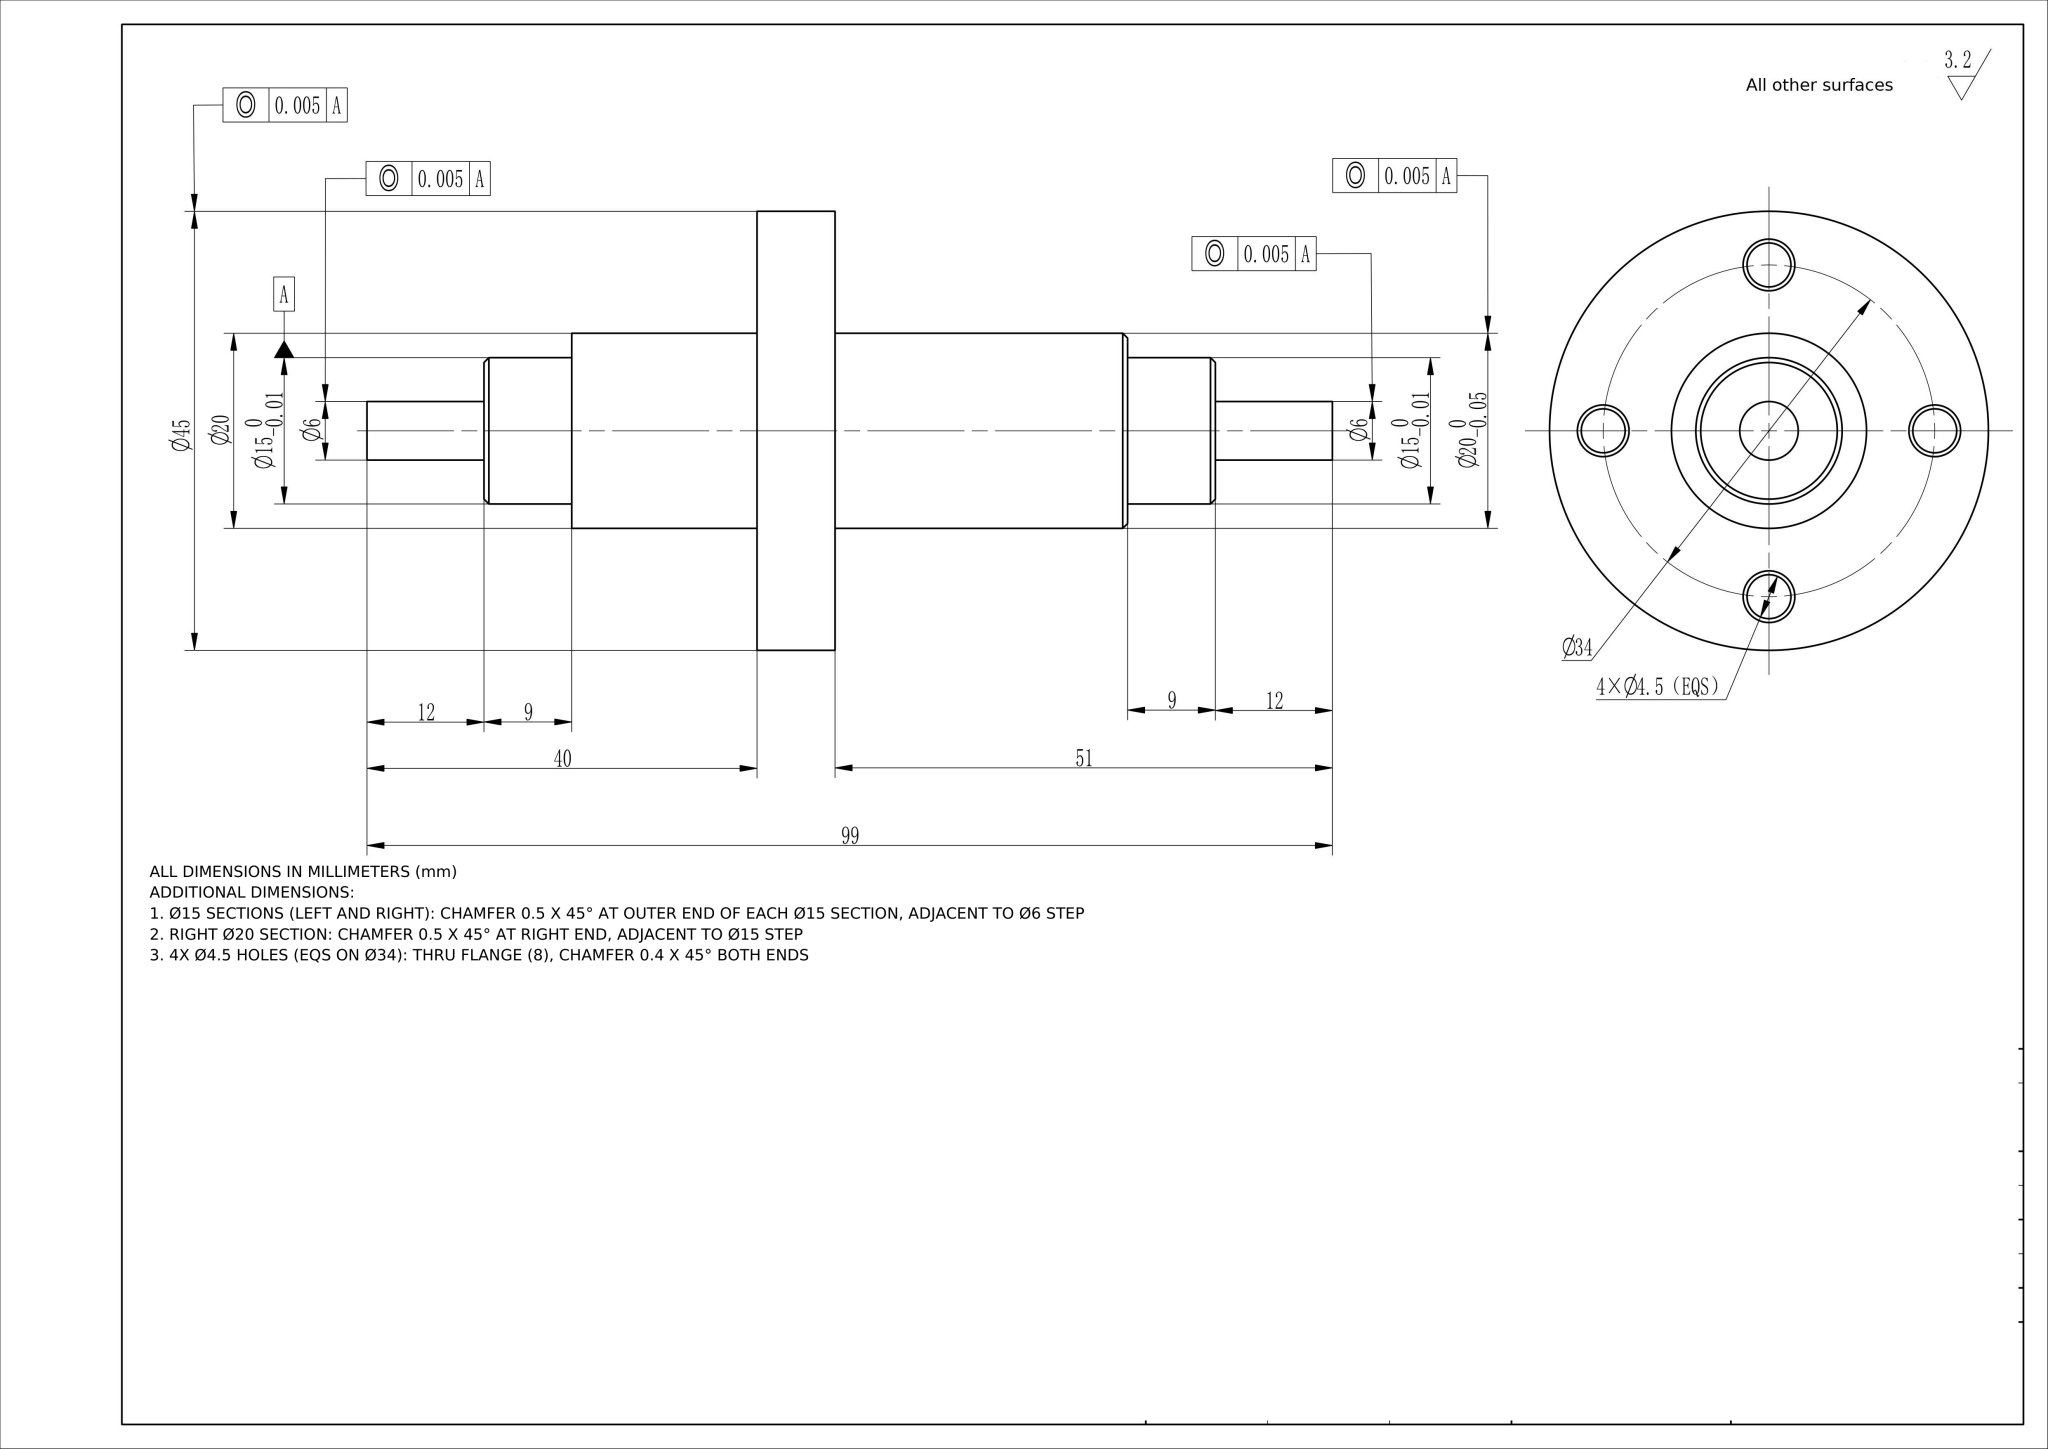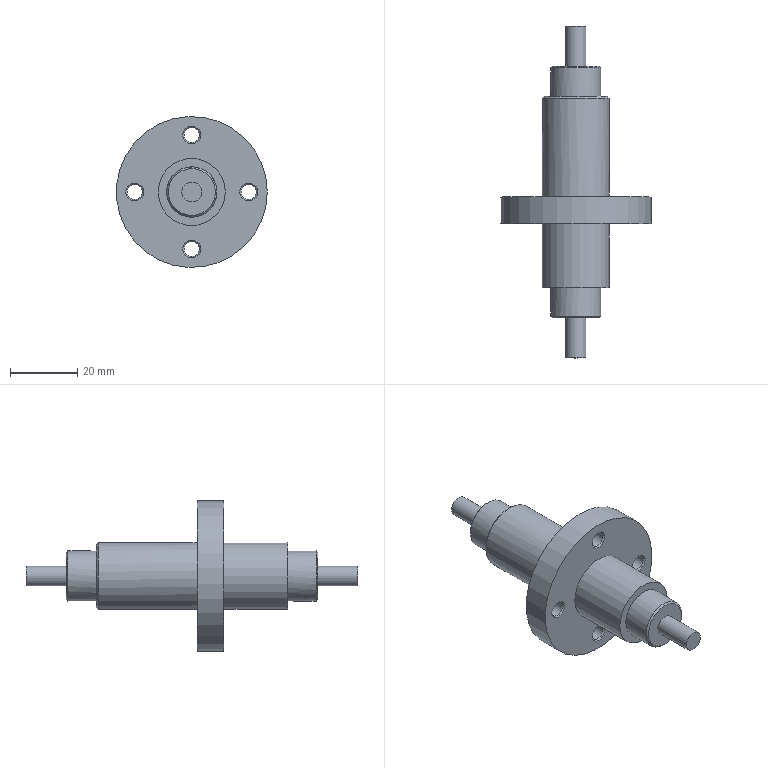Part | NX | mm | 1 solid | 30 faces | box 45 x 99 x 45 mm | volume 31439 mm3 | cylinder 11 | cone 11 | plane 8 | commonest cylinder face diameters 4.5 x4 20 x2 15 x2 6 x2 45 x1
STEP:
#1=CARTESIAN_POINT('',(0.,0.,0.));
#2=DIRECTION('',(0.,0.,1.));
#3=DIRECTION('',(1.,0.,0.));
#4=AXIS2_PLACEMENT_3D('',#1,#2,#3);
#5=(LENGTH_UNIT()NAMED_UNIT(*)SI_UNIT(.MILLI.,.METRE.));
#6=UNCERTAINTY_MEASURE_WITH_UNIT(LENGTH_MEASURE(0.00002),#5,'','');
#7=(NAMED_UNIT(*)PLANE_ANGLE_UNIT()SI_UNIT($,.RADIAN.));
#8=PLANE_ANGLE_MEASURE_WITH_UNIT(PLANE_ANGLE_MEASURE(0.01745),#7);
#9=DIMENSIONAL_EXPONENTS(0.,0.,0.,0.,0.,0.,0.);
#10=(CONVERSION_BASED_UNIT('',#8)NAMED_UNIT(#9)PLANE_ANGLE_UNIT());
#11=(NAMED_UNIT(*)SI_UNIT($,.STERADIAN.)SOLID_ANGLE_UNIT());
#12=(GEOMETRIC_REPRESENTATION_CONTEXT(3)GLOBAL_UNCERTAINTY_ASSIGNED_CONTEXT((#6))GLOBAL_UNIT_ASSIGNED_CONTEXT((#5,#10,#11))REPRESENTATION_CONTEXT('',''));
#13=SHAPE_REPRESENTATION('',(#4),#12);
#14=CARTESIAN_POINT('',(0.,29.5,-10.));
#15=VERTEX_POINT('',#14);
#16=CARTESIAN_POINT('',(0.,29.5,0.));
#17=DIRECTION('',(0.,-1.,0.));
#18=DIRECTION('',(0.,0.,-1.));
#19=AXIS2_PLACEMENT_3D('',#16,#17,#18);
#20=CIRCLE('',#19,10.);
#21=EDGE_CURVE('',#15,#15,#20,.T.);
#22=ORIENTED_EDGE('',*,*,#21,.T.);
#23=EDGE_LOOP('',(#22));
#24=FACE_BOUND('',#23,.T.);
#25=CARTESIAN_POINT('',(10.,0.,-0.));
#26=VERTEX_POINT('',#25);
#27=CARTESIAN_POINT('',(0.,0.,0.));
#28=DIRECTION('',(0.,-1.,0.));
#29=DIRECTION('',(1.,0.,-0.));
#30=AXIS2_PLACEMENT_3D('',#27,#28,#29);
#31=CIRCLE('',#30,10.);
#32=EDGE_CURVE('',#26,#26,#31,.T.);
#33=ORIENTED_EDGE('',*,*,#32,.F.);
#34=EDGE_LOOP('',(#33));
#35=FACE_BOUND('',#34,.T.);
#36=CARTESIAN_POINT('',(0.,30.,0.));
#37=DIRECTION('',(0.,-1.,0.));
#38=DIRECTION('',(0.,0.,-1.));
#39=AXIS2_PLACEMENT_3D('',#36,#37,#38);
#40=CYLINDRICAL_SURFACE('',#39,10.);
#41=ADVANCED_FACE('',(#24,#35),#40,.T.);
#42=CARTESIAN_POINT('',(0.,30.,-9.5));
#43=VERTEX_POINT('',#42);
#44=CARTESIAN_POINT('',(0.,30.,0.));
#45=DIRECTION('',(0.,1.,0.));
#46=DIRECTION('',(0.,0.,-1.));
#47=AXIS2_PLACEMENT_3D('',#44,#45,#46);
#48=CIRCLE('',#47,9.5);
#49=EDGE_CURVE('',#43,#43,#48,.T.);
#50=ORIENTED_EDGE('',*,*,#49,.T.);
#51=EDGE_LOOP('',(#50));
#52=FACE_BOUND('',#51,.T.);
#53=CARTESIAN_POINT('',(7.5,30.,0.));
#54=VERTEX_POINT('',#53);
#55=CARTESIAN_POINT('',(0.,30.,0.));
#56=DIRECTION('',(0.,1.,0.));
#57=DIRECTION('',(1.,0.,0.));
#58=AXIS2_PLACEMENT_3D('',#55,#56,#57);
#59=CIRCLE('',#58,7.5);
#60=EDGE_CURVE('',#54,#54,#59,.T.);
#61=ORIENTED_EDGE('',*,*,#60,.F.);
#62=EDGE_LOOP('',(#61));
#63=FACE_BOUND('',#62,.T.);
#64=CARTESIAN_POINT('',(0.,30.,0.));
#65=DIRECTION('',(0.,-1.,0.));
#66=DIRECTION('',(0.,0.,-1.));
#67=AXIS2_PLACEMENT_3D('',#64,#65,#66);
#68=PLANE('',#67);
#69=ADVANCED_FACE('',(#52,#63),#68,.F.);
#70=CARTESIAN_POINT('',(22.5,-8.,-0.));
#71=VERTEX_POINT('',#70);
#72=CARTESIAN_POINT('',(0.,-8.,0.));
#73=DIRECTION('',(0.,-1.,0.));
#74=DIRECTION('',(1.,0.,-0.));
#75=AXIS2_PLACEMENT_3D('',#72,#73,#74);
#76=CIRCLE('',#75,22.5);
#77=EDGE_CURVE('',#71,#71,#76,.T.);
#78=ORIENTED_EDGE('',*,*,#77,.F.);
#79=EDGE_LOOP('',(#78));
#80=FACE_BOUND('',#79,.T.);
#81=CARTESIAN_POINT('',(22.5,0.,-0.));
#82=VERTEX_POINT('',#81);
#83=CARTESIAN_POINT('',(0.,0.,0.));
#84=DIRECTION('',(0.,-1.,0.));
#85=DIRECTION('',(1.,0.,-0.));
#86=AXIS2_PLACEMENT_3D('',#83,#84,#85);
#87=CIRCLE('',#86,22.5);
#88=EDGE_CURVE('',#82,#82,#87,.T.);
#89=ORIENTED_EDGE('',*,*,#88,.T.);
#90=EDGE_LOOP('',(#89));
#91=FACE_BOUND('',#90,.T.);
#92=CARTESIAN_POINT('',(0.,-8.,0.));
#93=DIRECTION('',(0.,1.,0.));
#94=DIRECTION('',(0.,0.,1.));
#95=AXIS2_PLACEMENT_3D('',#92,#93,#94);
#96=CYLINDRICAL_SURFACE('',#95,22.5);
#97=ADVANCED_FACE('',(#80,#91),#96,.T.);
#98=CARTESIAN_POINT('',(17.,-8.,-2.65));
#99=VERTEX_POINT('',#98);
#100=CARTESIAN_POINT('',(17.,-8.,0.));
#101=DIRECTION('',(0.,1.,0.));
#102=DIRECTION('',(0.,0.,-1.));
#103=AXIS2_PLACEMENT_3D('',#100,#101,#102);
#104=CIRCLE('',#103,2.65);
#105=EDGE_CURVE('',#99,#99,#104,.T.);
#106=ORIENTED_EDGE('',*,*,#105,.T.);
#107=EDGE_LOOP('',(#106));
#108=FACE_BOUND('',#107,.T.);
#109=CARTESIAN_POINT('',(0.,-8.,14.35));
#110=VERTEX_POINT('',#109);
#111=CARTESIAN_POINT('',(0.,-8.,17.));
#112=DIRECTION('',(0.,1.,0.));
#113=DIRECTION('',(0.,0.,-1.));
#114=AXIS2_PLACEMENT_3D('',#111,#112,#113);
#115=CIRCLE('',#114,2.65);
#116=EDGE_CURVE('',#110,#110,#115,.T.);
#117=ORIENTED_EDGE('',*,*,#116,.T.);
#118=EDGE_LOOP('',(#117));
#119=FACE_BOUND('',#118,.T.);
#120=CARTESIAN_POINT('',(0.,-8.,-19.65));
#121=VERTEX_POINT('',#120);
#122=CARTESIAN_POINT('',(0.,-8.,-17.));
#123=DIRECTION('',(0.,1.,0.));
#124=DIRECTION('',(0.,0.,-1.));
#125=AXIS2_PLACEMENT_3D('',#122,#123,#124);
#126=CIRCLE('',#125,2.65);
#127=EDGE_CURVE('',#121,#121,#126,.T.);
#128=ORIENTED_EDGE('',*,*,#127,.T.);
#129=EDGE_LOOP('',(#128));
#130=FACE_BOUND('',#129,.T.);
#131=CARTESIAN_POINT('',(-17.,-8.,-2.65));
#132=VERTEX_POINT('',#131);
#133=CARTESIAN_POINT('',(-17.,-8.,0.));
#134=DIRECTION('',(0.,1.,0.));
#135=DIRECTION('',(0.,0.,-1.));
#136=AXIS2_PLACEMENT_3D('',#133,#134,#135);
#137=CIRCLE('',#136,2.65);
#138=EDGE_CURVE('',#132,#132,#137,.T.);
#139=ORIENTED_EDGE('',*,*,#138,.T.);
#140=EDGE_LOOP('',(#139));
#141=FACE_BOUND('',#140,.T.);
#142=CARTESIAN_POINT('',(10.,-8.,-0.));
#143=VERTEX_POINT('',#142);
#144=CARTESIAN_POINT('',(0.,-8.,0.));
#145=DIRECTION('',(0.,-1.,0.));
#146=DIRECTION('',(1.,0.,-0.));
#147=AXIS2_PLACEMENT_3D('',#144,#145,#146);
#148=CIRCLE('',#147,10.);
#149=EDGE_CURVE('',#143,#143,#148,.T.);
#150=ORIENTED_EDGE('',*,*,#149,.F.);
#151=EDGE_LOOP('',(#150));
#152=FACE_BOUND('',#151,.T.);
#153=ORIENTED_EDGE('',*,*,#77,.T.);
#154=EDGE_LOOP('',(#153));
#155=FACE_BOUND('',#154,.T.);
#156=CARTESIAN_POINT('',(0.,-8.,0.));
#157=DIRECTION('',(0.,-1.,0.));
#158=DIRECTION('',(0.,0.,-1.));
#159=AXIS2_PLACEMENT_3D('',#156,#157,#158);
#160=PLANE('',#159);
#161=ADVANCED_FACE('',(#108,#119,#130,#141,#152,#155),#160,.T.);
#162=CARTESIAN_POINT('',(17.,0.,-2.65));
#163=VERTEX_POINT('',#162);
#164=CARTESIAN_POINT('',(17.,0.,0.));
#165=DIRECTION('',(0.,-1.,0.));
#166=DIRECTION('',(0.,0.,-1.));
#167=AXIS2_PLACEMENT_3D('',#164,#165,#166);
#168=CIRCLE('',#167,2.65);
#169=EDGE_CURVE('',#163,#163,#168,.T.);
#170=ORIENTED_EDGE('',*,*,#169,.T.);
#171=EDGE_LOOP('',(#170));
#172=FACE_BOUND('',#171,.T.);
#173=CARTESIAN_POINT('',(0.,0.,14.35));
#174=VERTEX_POINT('',#173);
#175=CARTESIAN_POINT('',(0.,0.,17.));
#176=DIRECTION('',(0.,-1.,0.));
#177=DIRECTION('',(0.,0.,-1.));
#178=AXIS2_PLACEMENT_3D('',#175,#176,#177);
#179=CIRCLE('',#178,2.65);
#180=EDGE_CURVE('',#174,#174,#179,.T.);
#181=ORIENTED_EDGE('',*,*,#180,.T.);
#182=EDGE_LOOP('',(#181));
#183=FACE_BOUND('',#182,.T.);
#184=CARTESIAN_POINT('',(0.,0.,-19.65));
#185=VERTEX_POINT('',#184);
#186=CARTESIAN_POINT('',(0.,0.,-17.));
#187=DIRECTION('',(0.,-1.,0.));
#188=DIRECTION('',(0.,0.,-1.));
#189=AXIS2_PLACEMENT_3D('',#186,#187,#188);
#190=CIRCLE('',#189,2.65);
#191=EDGE_CURVE('',#185,#185,#190,.T.);
#192=ORIENTED_EDGE('',*,*,#191,.T.);
#193=EDGE_LOOP('',(#192));
#194=FACE_BOUND('',#193,.T.);
#195=CARTESIAN_POINT('',(-17.,0.,-2.65));
#196=VERTEX_POINT('',#195);
#197=CARTESIAN_POINT('',(-17.,0.,0.));
#198=DIRECTION('',(0.,-1.,0.));
#199=DIRECTION('',(0.,0.,-1.));
#200=AXIS2_PLACEMENT_3D('',#197,#198,#199);
#201=CIRCLE('',#200,2.65);
#202=EDGE_CURVE('',#196,#196,#201,.T.);
#203=ORIENTED_EDGE('',*,*,#202,.T.);
#204=EDGE_LOOP('',(#203));
#205=FACE_BOUND('',#204,.T.);
#206=ORIENTED_EDGE('',*,*,#32,.T.);
#207=EDGE_LOOP('',(#206));
#208=FACE_BOUND('',#207,.T.);
#209=ORIENTED_EDGE('',*,*,#88,.F.);
#210=EDGE_LOOP('',(#209));
#211=FACE_BOUND('',#210,.T.);
#212=CARTESIAN_POINT('',(0.,0.,0.));
#213=DIRECTION('',(0.,-1.,0.));
#214=DIRECTION('',(0.,0.,-1.));
#215=AXIS2_PLACEMENT_3D('',#212,#213,#214);
#216=PLANE('',#215);
#217=ADVANCED_FACE('',(#172,#183,#194,#205,#208,#211),#216,.F.);
#218=CARTESIAN_POINT('',(0.,38.5,7.5));
#219=VERTEX_POINT('',#218);
#220=CARTESIAN_POINT('',(0.,38.5,0.));
#221=DIRECTION('',(0.,-1.,0.));
#222=DIRECTION('',(0.,0.,1.));
#223=AXIS2_PLACEMENT_3D('',#220,#221,#222);
#224=CIRCLE('',#223,7.5);
#225=EDGE_CURVE('',#219,#219,#224,.T.);
#226=ORIENTED_EDGE('',*,*,#225,.T.);
#227=EDGE_LOOP('',(#226));
#228=FACE_BOUND('',#227,.T.);
#229=ORIENTED_EDGE('',*,*,#60,.T.);
#230=EDGE_LOOP('',(#229));
#231=FACE_BOUND('',#230,.T.);
#232=CARTESIAN_POINT('',(0.,39.,0.));
#233=DIRECTION('',(0.,-1.,0.));
#234=DIRECTION('',(0.,0.,-1.));
#235=AXIS2_PLACEMENT_3D('',#232,#233,#234);
#236=CYLINDRICAL_SURFACE('',#235,7.5);
#237=ADVANCED_FACE('',(#228,#231),#236,.T.);
#238=CARTESIAN_POINT('',(0.,39.,7.));
#239=VERTEX_POINT('',#238);
#240=CARTESIAN_POINT('',(0.,39.,0.));
#241=DIRECTION('',(0.,1.,0.));
#242=DIRECTION('',(0.,0.,1.));
#243=AXIS2_PLACEMENT_3D('',#240,#241,#242);
#244=CIRCLE('',#243,7.);
#245=EDGE_CURVE('',#239,#239,#244,.T.);
#246=ORIENTED_EDGE('',*,*,#245,.T.);
#247=EDGE_LOOP('',(#246));
#248=FACE_BOUND('',#247,.T.);
#249=CARTESIAN_POINT('',(3.,39.,0.));
#250=VERTEX_POINT('',#249);
#251=CARTESIAN_POINT('',(0.,39.,0.));
#252=DIRECTION('',(0.,1.,0.));
#253=DIRECTION('',(1.,0.,0.));
#254=AXIS2_PLACEMENT_3D('',#251,#252,#253);
#255=CIRCLE('',#254,3.);
#256=EDGE_CURVE('',#250,#250,#255,.T.);
#257=ORIENTED_EDGE('',*,*,#256,.F.);
#258=EDGE_LOOP('',(#257));
#259=FACE_BOUND('',#258,.T.);
#260=CARTESIAN_POINT('',(0.,39.,0.));
#261=DIRECTION('',(0.,1.,0.));
#262=DIRECTION('',(0.,0.,1.));
#263=AXIS2_PLACEMENT_3D('',#260,#261,#262);
#264=PLANE('',#263);
#265=ADVANCED_FACE('',(#248,#259),#264,.T.);
#266=CARTESIAN_POINT('',(10.,-27.,-0.));
#267=VERTEX_POINT('',#266);
#268=CARTESIAN_POINT('',(0.,-27.,0.));
#269=DIRECTION('',(0.,-1.,0.));
#270=DIRECTION('',(1.,0.,-0.));
#271=AXIS2_PLACEMENT_3D('',#268,#269,#270);
#272=CIRCLE('',#271,10.);
#273=EDGE_CURVE('',#267,#267,#272,.T.);
#274=ORIENTED_EDGE('',*,*,#273,.F.);
#275=EDGE_LOOP('',(#274));
#276=FACE_BOUND('',#275,.T.);
#277=ORIENTED_EDGE('',*,*,#149,.T.);
#278=EDGE_LOOP('',(#277));
#279=FACE_BOUND('',#278,.T.);
#280=CARTESIAN_POINT('',(0.,-27.,0.));
#281=DIRECTION('',(0.,1.,0.));
#282=DIRECTION('',(0.,0.,1.));
#283=AXIS2_PLACEMENT_3D('',#280,#281,#282);
#284=CYLINDRICAL_SURFACE('',#283,10.);
#285=ADVANCED_FACE('',(#276,#279),#284,.T.);
#286=CARTESIAN_POINT('',(7.5,-27.,-0.));
#287=VERTEX_POINT('',#286);
#288=CARTESIAN_POINT('',(0.,-27.,0.));
#289=DIRECTION('',(0.,-1.,0.));
#290=DIRECTION('',(1.,0.,-0.));
#291=AXIS2_PLACEMENT_3D('',#288,#289,#290);
#292=CIRCLE('',#291,7.5);
#293=EDGE_CURVE('',#287,#287,#292,.T.);
#294=ORIENTED_EDGE('',*,*,#293,.F.);
#295=EDGE_LOOP('',(#294));
#296=FACE_BOUND('',#295,.T.);
#297=ORIENTED_EDGE('',*,*,#273,.T.);
#298=EDGE_LOOP('',(#297));
#299=FACE_BOUND('',#298,.T.);
#300=CARTESIAN_POINT('',(0.,-27.,0.));
#301=DIRECTION('',(0.,-1.,0.));
#302=DIRECTION('',(0.,0.,-1.));
#303=AXIS2_PLACEMENT_3D('',#300,#301,#302);
#304=PLANE('',#303);
#305=ADVANCED_FACE('',(#296,#299),#304,.T.);
#306=CARTESIAN_POINT('',(0.,-35.5,-7.5));
#307=VERTEX_POINT('',#306);
#308=CARTESIAN_POINT('',(0.,-35.5,0.));
#309=DIRECTION('',(0.,1.,0.));
#310=DIRECTION('',(0.,0.,-1.));
#311=AXIS2_PLACEMENT_3D('',#308,#309,#310);
#312=CIRCLE('',#311,7.5);
#313=EDGE_CURVE('',#307,#307,#312,.T.);
#314=ORIENTED_EDGE('',*,*,#313,.T.);
#315=EDGE_LOOP('',(#314));
#316=FACE_BOUND('',#315,.T.);
#317=ORIENTED_EDGE('',*,*,#293,.T.);
#318=EDGE_LOOP('',(#317));
#319=FACE_BOUND('',#318,.T.);
#320=CARTESIAN_POINT('',(0.,-36.,0.));
#321=DIRECTION('',(0.,1.,0.));
#322=DIRECTION('',(0.,0.,1.));
#323=AXIS2_PLACEMENT_3D('',#320,#321,#322);
#324=CYLINDRICAL_SURFACE('',#323,7.5);
#325=ADVANCED_FACE('',(#316,#319),#324,.T.);
#326=CARTESIAN_POINT('',(0.,-36.,-7.));
#327=VERTEX_POINT('',#326);
#328=CARTESIAN_POINT('',(0.,-36.,0.));
#329=DIRECTION('',(0.,-1.,0.));
#330=DIRECTION('',(0.,0.,-1.));
#331=AXIS2_PLACEMENT_3D('',#328,#329,#330);
#332=CIRCLE('',#331,7.);
#333=EDGE_CURVE('',#327,#327,#332,.T.);
#334=ORIENTED_EDGE('',*,*,#333,.T.);
#335=EDGE_LOOP('',(#334));
#336=FACE_BOUND('',#335,.T.);
#337=CARTESIAN_POINT('',(3.,-36.,-0.));
#338=VERTEX_POINT('',#337);
#339=CARTESIAN_POINT('',(0.,-36.,0.));
#340=DIRECTION('',(0.,-1.,0.));
#341=DIRECTION('',(1.,0.,-0.));
#342=AXIS2_PLACEMENT_3D('',#339,#340,#341);
#343=CIRCLE('',#342,3.);
#344=EDGE_CURVE('',#338,#338,#343,.T.);
#345=ORIENTED_EDGE('',*,*,#344,.F.);
#346=EDGE_LOOP('',(#345));
#347=FACE_BOUND('',#346,.T.);
#348=CARTESIAN_POINT('',(0.,-36.,0.));
#349=DIRECTION('',(0.,-1.,0.));
#350=DIRECTION('',(0.,0.,-1.));
#351=AXIS2_PLACEMENT_3D('',#348,#349,#350);
#352=PLANE('',#351);
#353=ADVANCED_FACE('',(#336,#347),#352,.T.);
#354=CARTESIAN_POINT('',(-17.,-0.4,-2.25));
#355=VERTEX_POINT('',#354);
#356=CARTESIAN_POINT('',(-17.,-0.4,0.));
#357=DIRECTION('',(0.,1.,0.));
#358=DIRECTION('',(0.,0.,-1.));
#359=AXIS2_PLACEMENT_3D('',#356,#357,#358);
#360=CIRCLE('',#359,2.25);
#361=EDGE_CURVE('',#355,#355,#360,.T.);
#362=ORIENTED_EDGE('',*,*,#361,.T.);
#363=EDGE_LOOP('',(#362));
#364=FACE_BOUND('',#363,.T.);
#365=CARTESIAN_POINT('',(-17.,-7.6,-2.25));
#366=VERTEX_POINT('',#365);
#367=CARTESIAN_POINT('',(-17.,-7.6,0.));
#368=DIRECTION('',(0.,-1.,0.));
#369=DIRECTION('',(0.,0.,-1.));
#370=AXIS2_PLACEMENT_3D('',#367,#368,#369);
#371=CIRCLE('',#370,2.25);
#372=EDGE_CURVE('',#366,#366,#371,.T.);
#373=ORIENTED_EDGE('',*,*,#372,.T.);
#374=EDGE_LOOP('',(#373));
#375=FACE_BOUND('',#374,.T.);
#376=CARTESIAN_POINT('',(-17.,-8.,0.));
#377=DIRECTION('',(0.,1.,0.));
#378=DIRECTION('',(0.,0.,1.));
#379=AXIS2_PLACEMENT_3D('',#376,#377,#378);
#380=CYLINDRICAL_SURFACE('',#379,2.25);
#381=ADVANCED_FACE('',(#364,#375),#380,.F.);
#382=ORIENTED_EDGE('',*,*,#372,.F.);
#383=EDGE_LOOP('',(#382));
#384=FACE_BOUND('',#383,.T.);
#385=ORIENTED_EDGE('',*,*,#138,.F.);
#386=EDGE_LOOP('',(#385));
#387=FACE_BOUND('',#386,.T.);
#388=CARTESIAN_POINT('',(-17.,-8.,0.));
#389=DIRECTION('',(0.,-1.,0.));
#390=DIRECTION('',(0.,0.,-1.));
#391=AXIS2_PLACEMENT_3D('',#388,#389,#390);
#392=CONICAL_SURFACE('',#391,2.65,45.);
#393=ADVANCED_FACE('',(#384,#387),#392,.F.);
#394=ORIENTED_EDGE('',*,*,#202,.F.);
#395=EDGE_LOOP('',(#394));
#396=FACE_BOUND('',#395,.T.);
#397=ORIENTED_EDGE('',*,*,#361,.F.);
#398=EDGE_LOOP('',(#397));
#399=FACE_BOUND('',#398,.T.);
#400=CARTESIAN_POINT('',(-17.,-0.4,0.));
#401=DIRECTION('',(0.,1.,0.));
#402=DIRECTION('',(0.,0.,1.));
#403=AXIS2_PLACEMENT_3D('',#400,#401,#402);
#404=CONICAL_SURFACE('',#403,2.25,45.);
#405=ADVANCED_FACE('',(#396,#399),#404,.F.);
#406=CARTESIAN_POINT('',(0.,-0.4,-19.25));
#407=VERTEX_POINT('',#406);
#408=CARTESIAN_POINT('',(0.,-0.4,-17.));
#409=DIRECTION('',(0.,1.,0.));
#410=DIRECTION('',(0.,0.,-1.));
#411=AXIS2_PLACEMENT_3D('',#408,#409,#410);
#412=CIRCLE('',#411,2.25);
#413=EDGE_CURVE('',#407,#407,#412,.T.);
#414=ORIENTED_EDGE('',*,*,#413,.T.);
#415=EDGE_LOOP('',(#414));
#416=FACE_BOUND('',#415,.T.);
#417=CARTESIAN_POINT('',(0.,-7.6,-19.25));
#418=VERTEX_POINT('',#417);
#419=CARTESIAN_POINT('',(0.,-7.6,-17.));
#420=DIRECTION('',(0.,-1.,0.));
#421=DIRECTION('',(0.,0.,-1.));
#422=AXIS2_PLACEMENT_3D('',#419,#420,#421);
#423=CIRCLE('',#422,2.25);
#424=EDGE_CURVE('',#418,#418,#423,.T.);
#425=ORIENTED_EDGE('',*,*,#424,.T.);
#426=EDGE_LOOP('',(#425));
#427=FACE_BOUND('',#426,.T.);
#428=CARTESIAN_POINT('',(0.,-8.,-17.));
#429=DIRECTION('',(0.,1.,0.));
#430=DIRECTION('',(0.,0.,1.));
#431=AXIS2_PLACEMENT_3D('',#428,#429,#430);
#432=CYLINDRICAL_SURFACE('',#431,2.25);
#433=ADVANCED_FACE('',(#416,#427),#432,.F.);
#434=ORIENTED_EDGE('',*,*,#424,.F.);
#435=EDGE_LOOP('',(#434));
#436=FACE_BOUND('',#435,.T.);
#437=ORIENTED_EDGE('',*,*,#127,.F.);
#438=EDGE_LOOP('',(#437));
#439=FACE_BOUND('',#438,.T.);
#440=CARTESIAN_POINT('',(0.,-8.,-17.));
#441=DIRECTION('',(0.,-1.,0.));
#442=DIRECTION('',(0.,0.,-1.));
#443=AXIS2_PLACEMENT_3D('',#440,#441,#442);
#444=CONICAL_SURFACE('',#443,2.65,45.);
#445=ADVANCED_FACE('',(#436,#439),#444,.F.);
#446=ORIENTED_EDGE('',*,*,#191,.F.);
#447=EDGE_LOOP('',(#446));
#448=FACE_BOUND('',#447,.T.);
#449=ORIENTED_EDGE('',*,*,#413,.F.);
#450=EDGE_LOOP('',(#449));
#451=FACE_BOUND('',#450,.T.);
#452=CARTESIAN_POINT('',(0.,-0.4,-17.));
#453=DIRECTION('',(0.,1.,0.));
#454=DIRECTION('',(0.,0.,1.));
#455=AXIS2_PLACEMENT_3D('',#452,#453,#454);
#456=CONICAL_SURFACE('',#455,2.25,45.);
#457=ADVANCED_FACE('',(#448,#451),#456,.F.);
#458=CARTESIAN_POINT('',(0.,-0.4,14.75));
#459=VERTEX_POINT('',#458);
#460=CARTESIAN_POINT('',(0.,-0.4,17.));
#461=DIRECTION('',(0.,1.,0.));
#462=DIRECTION('',(0.,0.,-1.));
#463=AXIS2_PLACEMENT_3D('',#460,#461,#462);
#464=CIRCLE('',#463,2.25);
#465=EDGE_CURVE('',#459,#459,#464,.T.);
#466=ORIENTED_EDGE('',*,*,#465,.T.);
#467=EDGE_LOOP('',(#466));
#468=FACE_BOUND('',#467,.T.);
#469=CARTESIAN_POINT('',(0.,-7.6,14.75));
#470=VERTEX_POINT('',#469);
#471=CARTESIAN_POINT('',(0.,-7.6,17.));
#472=DIRECTION('',(0.,-1.,0.));
#473=DIRECTION('',(0.,0.,-1.));
#474=AXIS2_PLACEMENT_3D('',#471,#472,#473);
#475=CIRCLE('',#474,2.25);
#476=EDGE_CURVE('',#470,#470,#475,.T.);
#477=ORIENTED_EDGE('',*,*,#476,.T.);
#478=EDGE_LOOP('',(#477));
#479=FACE_BOUND('',#478,.T.);
#480=CARTESIAN_POINT('',(0.,-8.,17.));
#481=DIRECTION('',(0.,1.,0.));
#482=DIRECTION('',(0.,0.,1.));
#483=AXIS2_PLACEMENT_3D('',#480,#481,#482);
#484=CYLINDRICAL_SURFACE('',#483,2.25);
#485=ADVANCED_FACE('',(#468,#479),#484,.F.);
#486=ORIENTED_EDGE('',*,*,#476,.F.);
#487=EDGE_LOOP('',(#486));
#488=FACE_BOUND('',#487,.T.);
#489=ORIENTED_EDGE('',*,*,#116,.F.);
#490=EDGE_LOOP('',(#489));
#491=FACE_BOUND('',#490,.T.);
#492=CARTESIAN_POINT('',(0.,-8.,17.));
#493=DIRECTION('',(0.,-1.,0.));
#494=DIRECTION('',(0.,0.,-1.));
#495=AXIS2_PLACEMENT_3D('',#492,#493,#494);
#496=CONICAL_SURFACE('',#495,2.65,45.);
#497=ADVANCED_FACE('',(#488,#491),#496,.F.);
#498=ORIENTED_EDGE('',*,*,#180,.F.);
#499=EDGE_LOOP('',(#498));
#500=FACE_BOUND('',#499,.T.);
#501=ORIENTED_EDGE('',*,*,#465,.F.);
#502=EDGE_LOOP('',(#501));
#503=FACE_BOUND('',#502,.T.);
#504=CARTESIAN_POINT('',(0.,-0.4,17.));
#505=DIRECTION('',(0.,1.,0.));
#506=DIRECTION('',(0.,0.,1.));
#507=AXIS2_PLACEMENT_3D('',#504,#505,#506);
#508=CONICAL_SURFACE('',#507,2.25,45.);
#509=ADVANCED_FACE('',(#500,#503),#508,.F.);
#510=CARTESIAN_POINT('',(17.,-0.4,-2.25));
#511=VERTEX_POINT('',#510);
#512=CARTESIAN_POINT('',(17.,-0.4,0.));
#513=DIRECTION('',(0.,1.,0.));
#514=DIRECTION('',(0.,0.,-1.));
#515=AXIS2_PLACEMENT_3D('',#512,#513,#514);
#516=CIRCLE('',#515,2.25);
#517=EDGE_CURVE('',#511,#511,#516,.T.);
#518=ORIENTED_EDGE('',*,*,#517,.T.);
#519=EDGE_LOOP('',(#518));
#520=FACE_BOUND('',#519,.T.);
#521=CARTESIAN_POINT('',(17.,-7.6,-2.25));
#522=VERTEX_POINT('',#521);
#523=CARTESIAN_POINT('',(17.,-7.6,0.));
#524=DIRECTION('',(0.,-1.,0.));
#525=DIRECTION('',(0.,0.,-1.));
#526=AXIS2_PLACEMENT_3D('',#523,#524,#525);
#527=CIRCLE('',#526,2.25);
#528=EDGE_CURVE('',#522,#522,#527,.T.);
#529=ORIENTED_EDGE('',*,*,#528,.T.);
#530=EDGE_LOOP('',(#529));
#531=FACE_BOUND('',#530,.T.);
#532=CARTESIAN_POINT('',(17.,-8.,0.));
#533=DIRECTION('',(0.,1.,0.));
#534=DIRECTION('',(0.,0.,1.));
#535=AXIS2_PLACEMENT_3D('',#532,#533,#534);
#536=CYLINDRICAL_SURFACE('',#535,2.25);
#537=ADVANCED_FACE('',(#520,#531),#536,.F.);
#538=ORIENTED_EDGE('',*,*,#528,.F.);
#539=EDGE_LOOP('',(#538));
#540=FACE_BOUND('',#539,.T.);
#541=ORIENTED_EDGE('',*,*,#105,.F.);
#542=EDGE_LOOP('',(#541));
#543=FACE_BOUND('',#542,.T.);
#544=CARTESIAN_POINT('',(17.,-8.,0.));
#545=DIRECTION('',(0.,-1.,0.));
#546=DIRECTION('',(0.,0.,-1.));
#547=AXIS2_PLACEMENT_3D('',#544,#545,#546);
#548=CONICAL_SURFACE('',#547,2.65,45.);
#549=ADVANCED_FACE('',(#540,#543),#548,.F.);
#550=ORIENTED_EDGE('',*,*,#169,.F.);
#551=EDGE_LOOP('',(#550));
#552=FACE_BOUND('',#551,.T.);
#553=ORIENTED_EDGE('',*,*,#517,.F.);
#554=EDGE_LOOP('',(#553));
#555=FACE_BOUND('',#554,.T.);
#556=CARTESIAN_POINT('',(17.,-0.4,0.));
#557=DIRECTION('',(0.,1.,0.));
#558=DIRECTION('',(0.,0.,1.));
#559=AXIS2_PLACEMENT_3D('',#556,#557,#558);
#560=CONICAL_SURFACE('',#559,2.25,45.);
#561=ADVANCED_FACE('',(#552,#555),#560,.F.);
#562=CARTESIAN_POINT('',(3.,-48.,-0.));
#563=VERTEX_POINT('',#562);
#564=CARTESIAN_POINT('',(0.,-48.,0.));
#565=DIRECTION('',(0.,-1.,0.));
#566=DIRECTION('',(1.,0.,-0.));
#567=AXIS2_PLACEMENT_3D('',#564,#565,#566);
#568=CIRCLE('',#567,3.);
#569=EDGE_CURVE('',#563,#563,#568,.T.);
#570=ORIENTED_EDGE('',*,*,#569,.F.);
#571=EDGE_LOOP('',(#570));
#572=FACE_BOUND('',#571,.T.);
#573=ORIENTED_EDGE('',*,*,#344,.T.);
#574=EDGE_LOOP('',(#573));
#575=FACE_BOUND('',#574,.T.);
#576=CARTESIAN_POINT('',(0.,-48.,0.));
#577=DIRECTION('',(0.,1.,0.));
#578=DIRECTION('',(0.,0.,1.));
#579=AXIS2_PLACEMENT_3D('',#576,#577,#578);
#580=CYLINDRICAL_SURFACE('',#579,3.);
#581=ADVANCED_FACE('',(#572,#575),#580,.T.);
#582=ORIENTED_EDGE('',*,*,#569,.T.);
#583=EDGE_LOOP('',(#582));
#584=FACE_OUTER_BOUND('',#583,.T.);
#585=CARTESIAN_POINT('',(0.,-48.,0.));
#586=DIRECTION('',(0.,-1.,0.));
#587=DIRECTION('',(0.,0.,-1.));
#588=AXIS2_PLACEMENT_3D('',#585,#586,#587);
#589=PLANE('',#588);
#590=ADVANCED_FACE('',(#584),#589,.T.);
#591=CARTESIAN_POINT('',(3.,51.,0.));
#592=VERTEX_POINT('',#591);
#593=CARTESIAN_POINT('',(0.,51.,0.));
#594=DIRECTION('',(0.,1.,0.));
#595=DIRECTION('',(1.,0.,0.));
#596=AXIS2_PLACEMENT_3D('',#593,#594,#595);
#597=CIRCLE('',#596,3.);
#598=EDGE_CURVE('',#592,#592,#597,.T.);
#599=ORIENTED_EDGE('',*,*,#598,.F.);
#600=EDGE_LOOP('',(#599));
#601=FACE_BOUND('',#600,.T.);
#602=ORIENTED_EDGE('',*,*,#256,.T.);
#603=EDGE_LOOP('',(#602));
#604=FACE_BOUND('',#603,.T.);
#605=CARTESIAN_POINT('',(0.,51.,0.));
#606=DIRECTION('',(0.,-1.,0.));
#607=DIRECTION('',(0.,0.,-1.));
#608=AXIS2_PLACEMENT_3D('',#605,#606,#607);
#609=CYLINDRICAL_SURFACE('',#608,3.);
#610=ADVANCED_FACE('',(#601,#604),#609,.T.);
#611=ORIENTED_EDGE('',*,*,#598,.T.);
#612=EDGE_LOOP('',(#611));
#613=FACE_OUTER_BOUND('',#612,.T.);
#614=CARTESIAN_POINT('',(0.,51.,0.));
#615=DIRECTION('',(0.,1.,0.));
#616=DIRECTION('',(0.,0.,1.));
#617=AXIS2_PLACEMENT_3D('',#614,#615,#616);
#618=PLANE('',#617);
#619=ADVANCED_FACE('',(#613),#618,.T.);
#620=ORIENTED_EDGE('',*,*,#49,.F.);
#621=EDGE_LOOP('',(#620));
#622=FACE_BOUND('',#621,.T.);
#623=ORIENTED_EDGE('',*,*,#21,.F.);
#624=EDGE_LOOP('',(#623));
#625=FACE_BOUND('',#624,.T.);
#626=CARTESIAN_POINT('',(0.,29.5,0.));
#627=DIRECTION('',(0.,-1.,0.));
#628=DIRECTION('',(0.,-0.,-1.));
#629=AXIS2_PLACEMENT_3D('',#626,#627,#628);
#630=CONICAL_SURFACE('',#629,10.,45.);
#631=ADVANCED_FACE('',(#622,#625),#630,.T.);
#632=ORIENTED_EDGE('',*,*,#313,.F.);
#633=EDGE_LOOP('',(#632));
#634=FACE_BOUND('',#633,.T.);
#635=ORIENTED_EDGE('',*,*,#333,.F.);
#636=EDGE_LOOP('',(#635));
#637=FACE_BOUND('',#636,.T.);
#638=CARTESIAN_POINT('',(0.,-36.,0.));
#639=DIRECTION('',(0.,1.,0.));
#640=DIRECTION('',(0.,-0.,1.));
#641=AXIS2_PLACEMENT_3D('',#638,#639,#640);
#642=CONICAL_SURFACE('',#641,7.,45.);
#643=ADVANCED_FACE('',(#634,#637),#642,.T.);
#644=ORIENTED_EDGE('',*,*,#225,.F.);
#645=EDGE_LOOP('',(#644));
#646=FACE_BOUND('',#645,.T.);
#647=ORIENTED_EDGE('',*,*,#245,.F.);
#648=EDGE_LOOP('',(#647));
#649=FACE_BOUND('',#648,.T.);
#650=CARTESIAN_POINT('',(0.,39.,0.));
#651=DIRECTION('',(0.,-1.,0.));
#652=DIRECTION('',(0.,0.,-1.));
#653=AXIS2_PLACEMENT_3D('',#650,#651,#652);
#654=CONICAL_SURFACE('',#653,7.,45.);
#655=ADVANCED_FACE('',(#646,#649),#654,.T.);
#656=CLOSED_SHELL('',(#41,#69,#97,#161,#217,#237,#265,#285,#305,#325,#353,#381,#393,#405,#433,#445,#457,#485,#497,#509,#537,#549,#561,#581,#590,#610,#619,#631,#643,#655));
#657=MANIFOLD_SOLID_BREP('',#656);
#658=ADVANCED_BREP_SHAPE_REPRESENTATION('',(#657),#12);
#659=SHAPE_REPRESENTATION_RELATIONSHIP('','',#13,#658);
#660=PRESENTATION_LAYER_ASSIGNMENT('','',(#657));
#661=COLOUR_RGB('',1.,0.6,0.);
#662=FILL_AREA_STYLE_COLOUR('',#661);
#663=FILL_AREA_STYLE('',(#662));
#664=SURFACE_STYLE_FILL_AREA(#663);
#665=SURFACE_SIDE_STYLE('',(#664));
#666=SURFACE_STYLE_USAGE(.BOTH.,#665);
#667=PRESENTATION_STYLE_ASSIGNMENT((#666));
#668=STYLED_ITEM('',(#667),#657);
#669=MECHANICAL_DESIGN_GEOMETRIC_PRESENTATION_REPRESENTATION('',(#668),#12);